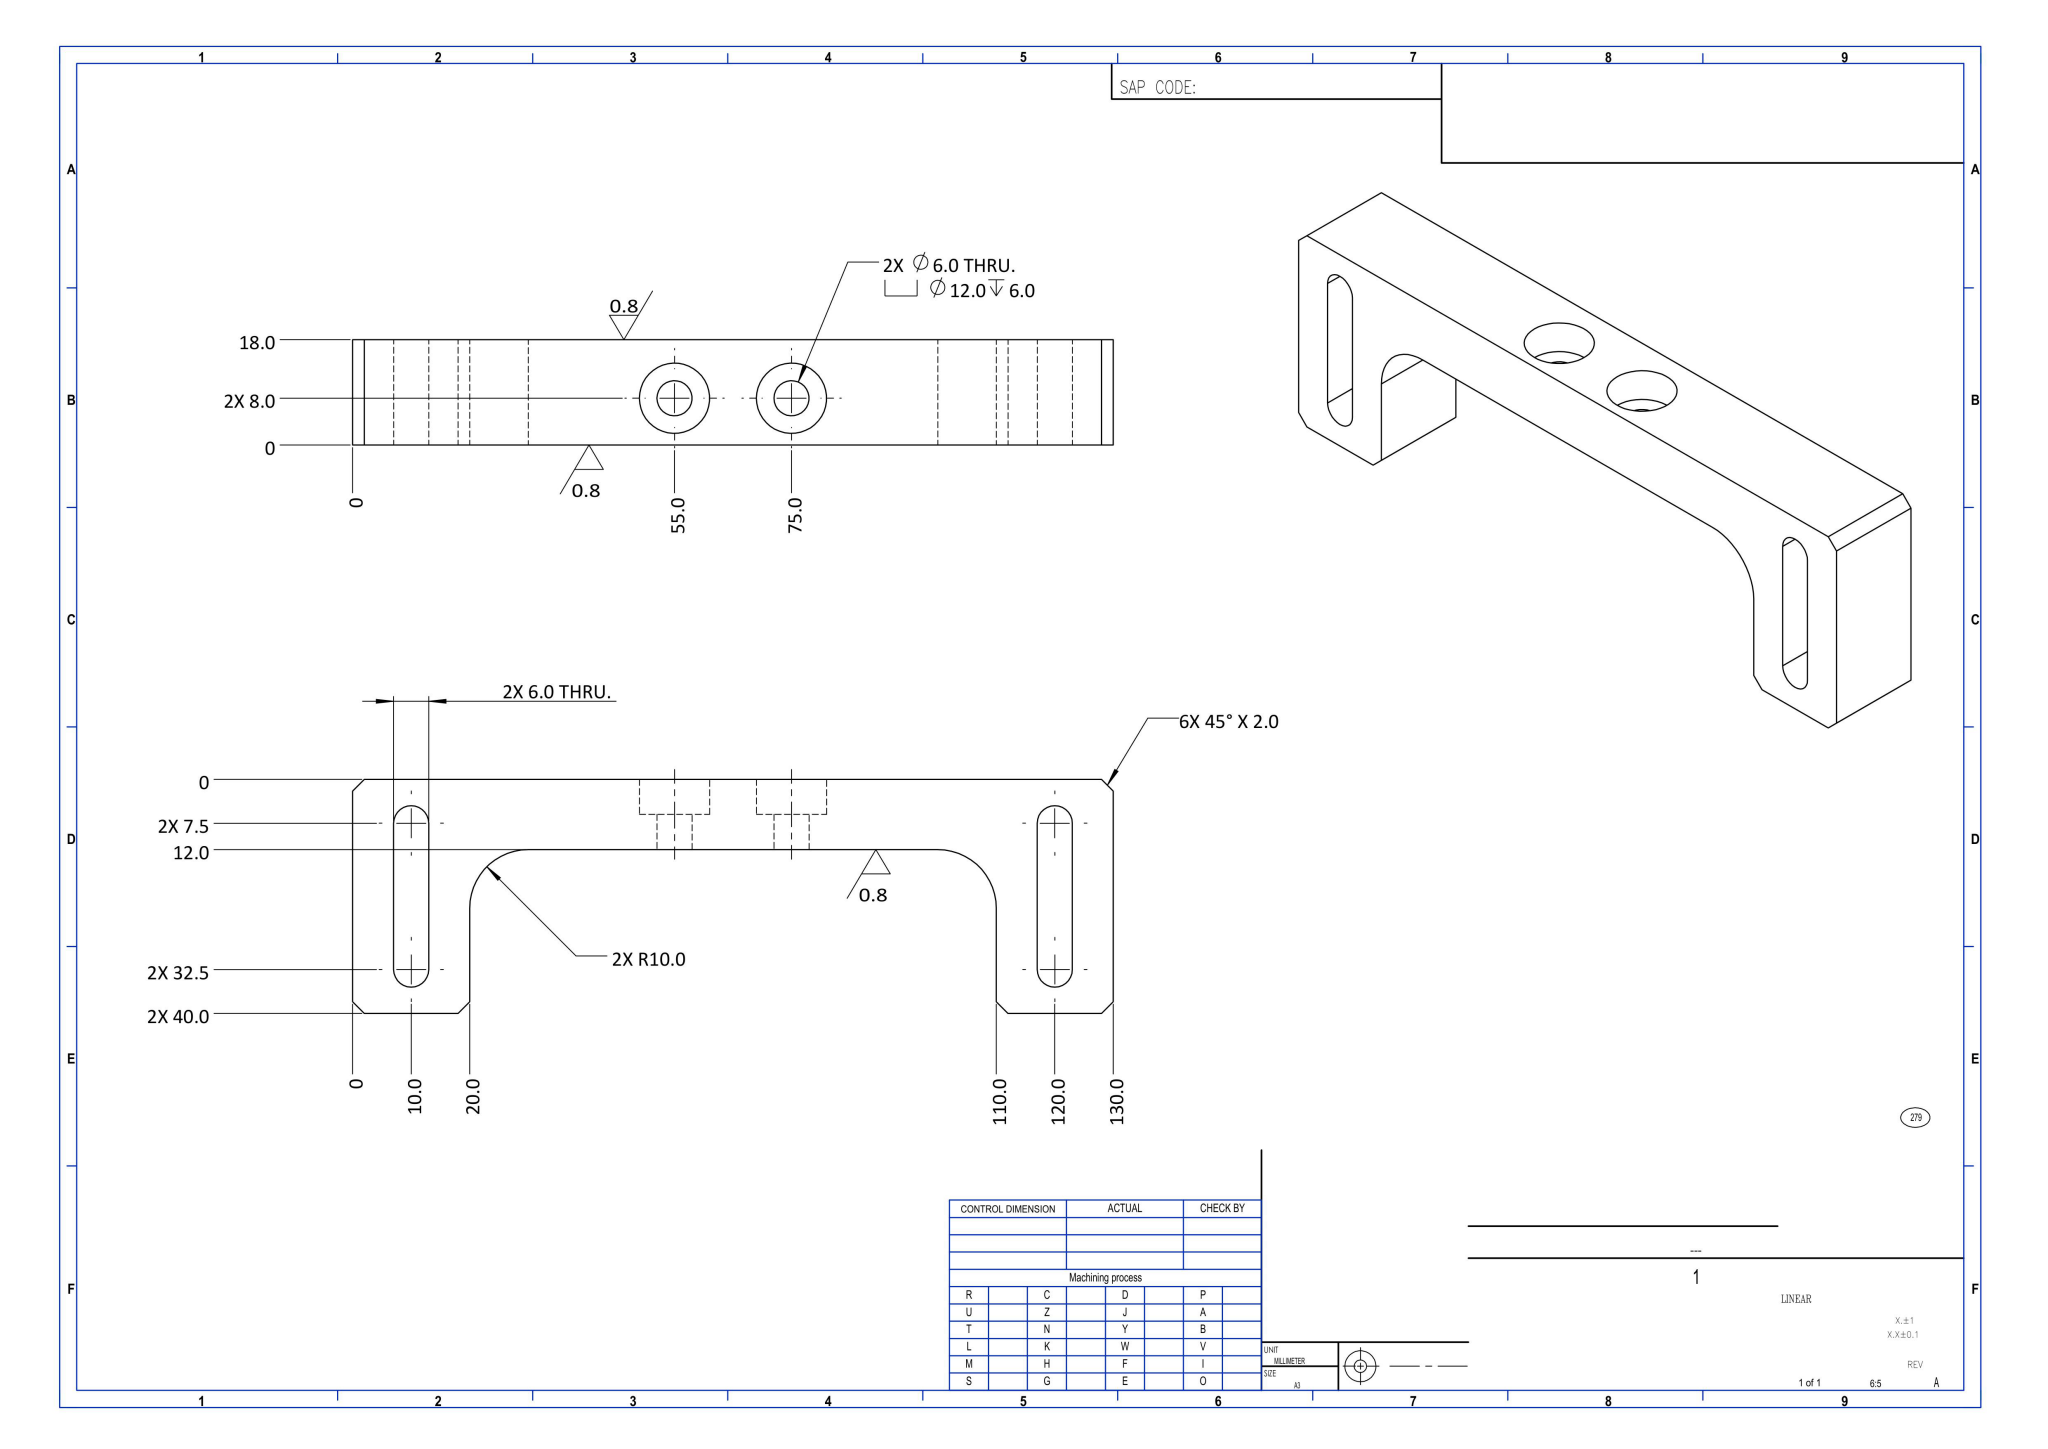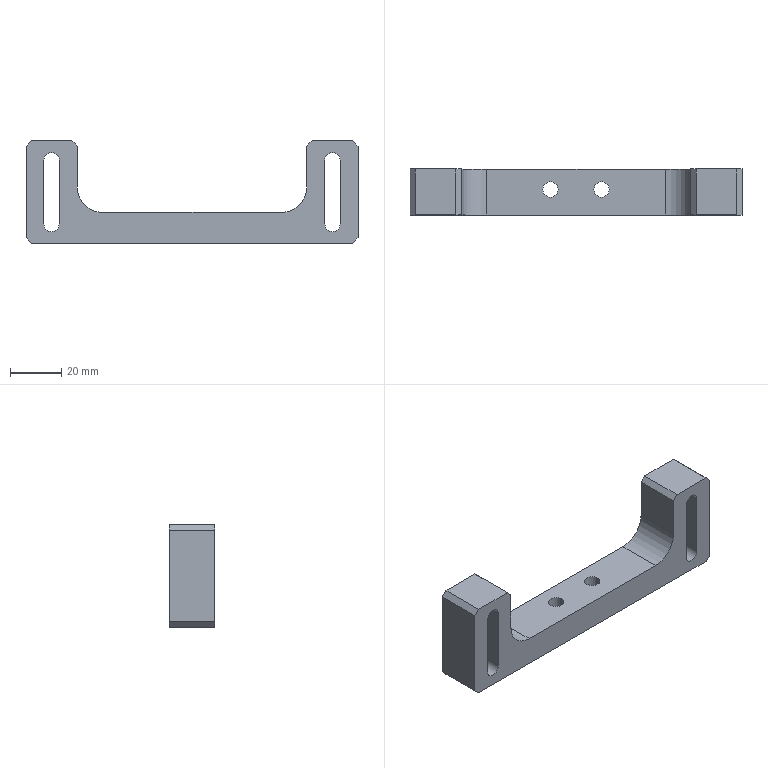Part | NX | mm | 1 solid | 38 faces | box 130 x 18 x 40 mm | volume 40682 mm3 | plane 22 | cylinder 16 | commonest cylinder face diameters 6 x10 12 x4 20 x2